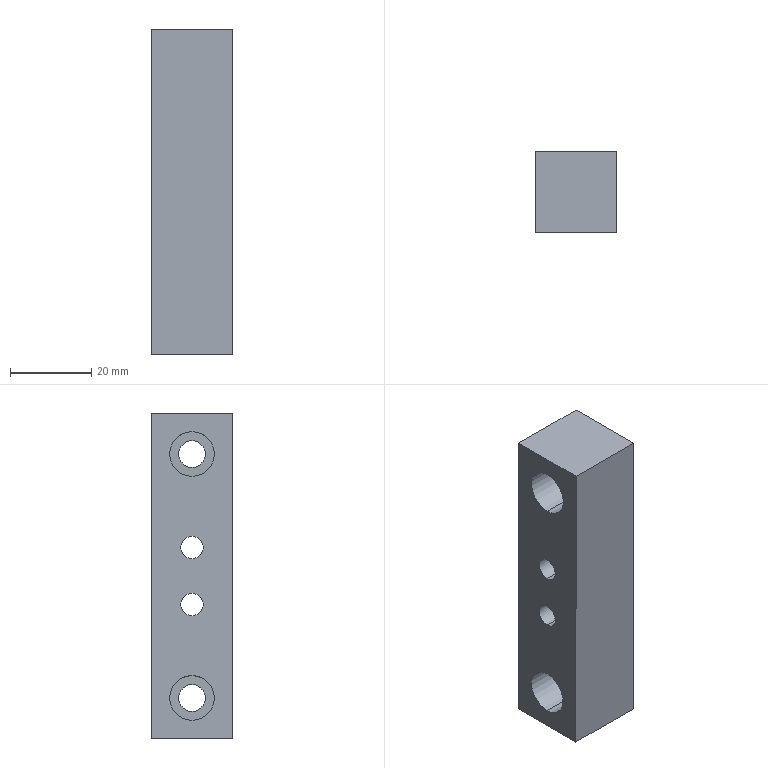Component | SolidWorks | ArmRotationCylinderConnectionBlock-1 | 1 solid | 26 faces | box 20.09 x 20 x 80.02 mm | volume 27354 mm3 | cylinder 16 | plane 10 | commonest cylinder face diameters 10 x4 5.5 x4 11 x4 6.6 x4
build123d program:
from build123d import *

# Parameters (mm, degrees)
SKETCH1_W                                       = 20
SKETCH1_H                                       = 80
BOSS_EXTRUDE1_DEPTH                             = 20
M6_HEX_SOCKET_HEAD_CAP_SCREW_CBORE1_D           = 6.6
M6_HEX_SOCKET_HEAD_CAP_SCREW_CBORE1_DEPTH       = 21
M6_HEX_SOCKET_HEAD_CAP_SCREW_CBORE1_CBORE_D     = 11
M6_HEX_SOCKET_HEAD_CAP_SCREW_CBORE1_CBORE_DEPTH = 14
M6_HEX_SOCKET_HEAD_CAP_SCREW_CBORE1_TIP         = 1.983
M5_HEX_SOCKET_HEAD_CAP_SCREW_CBORE1_D           = 5.5
M5_HEX_SOCKET_HEAD_CAP_SCREW_CBORE1_CBORE_D     = 10
M5_HEX_SOCKET_HEAD_CAP_SCREW_CBORE1_CBORE_DEPTH = 5.7


with BuildPart() as part:
    # Sketch1 → Boss-Extrude1 (new body)
    with BuildSketch(Plane(origin=(0, 0, 0), x_dir=(1, 0, 0), z_dir=(0, 1, 0))):
        Rectangle(SKETCH1_W, SKETCH1_H)
    extrude(amount=BOSS_EXTRUDE1_DEPTH)

    # M6 Hex Socket Head Cap Screw CBORE1
    with Locations(Plane.ZY.offset(10)):
        with Locations((-30, 10), (30, 10)):
            CounterBoreHole(M6_HEX_SOCKET_HEAD_CAP_SCREW_CBORE1_D / 2, M6_HEX_SOCKET_HEAD_CAP_SCREW_CBORE1_CBORE_D / 2, M6_HEX_SOCKET_HEAD_CAP_SCREW_CBORE1_CBORE_DEPTH, depth=M6_HEX_SOCKET_HEAD_CAP_SCREW_CBORE1_DEPTH)
            with Locations((0, 0, -(M6_HEX_SOCKET_HEAD_CAP_SCREW_CBORE1_DEPTH + M6_HEX_SOCKET_HEAD_CAP_SCREW_CBORE1_TIP / 2))):  # 118° drill point
                Cone(0, M6_HEX_SOCKET_HEAD_CAP_SCREW_CBORE1_D / 2, M6_HEX_SOCKET_HEAD_CAP_SCREW_CBORE1_TIP, mode=Mode.SUBTRACT)

    # M5 Hex Socket Head Cap Screw CBORE1 (through all)
    with Locations(Plane(origin=(10, 0, 0), x_dir=(0, 0, -1), z_dir=(1, 0, 0))):
        with Locations((-7, 10), (7, 10)):
            CounterBoreHole(M5_HEX_SOCKET_HEAD_CAP_SCREW_CBORE1_D / 2, M5_HEX_SOCKET_HEAD_CAP_SCREW_CBORE1_CBORE_D / 2, M5_HEX_SOCKET_HEAD_CAP_SCREW_CBORE1_CBORE_DEPTH)


solid = part.part

# Placed as in the assembly
solid = solid.moved(Location((-90.542, 904.54, 1109.715), (0, 0.0619, 0)))
STEP:
#1=COLOUR_RGB('',0.7922,0.8196,0.9333);
#2=FILL_AREA_STYLE_COLOUR('',#1);
#3=FILL_AREA_STYLE('',(#2));
#4=SURFACE_STYLE_FILL_AREA(#3);
#5=SURFACE_SIDE_STYLE('',(#4));
#6=SURFACE_STYLE_USAGE(.BOTH.,#5);
#7=PRESENTATION_STYLE_ASSIGNMENT((#6));
#8=CARTESIAN_POINT('',(-3.395,36.006,44.162));
#9=VERTEX_POINT('',#8);
#10=CARTESIAN_POINT('',(-3.395,36.006,43.768));
#11=VERTEX_POINT('',#10);
#12=CARTESIAN_POINT('',(-3.395,36.006,43.965));
#13=DIRECTION('',(1.,0.,-0.00108));
#14=DIRECTION('',(-0.00108,0.,-1.));
#15=AXIS2_PLACEMENT_3D('',#12,#13,#14);
#16=CIRCLE('',#15,0.1969);
#17=EDGE_CURVE('',#9,#11,#16,.T.);
#18=ORIENTED_EDGE('',*,*,#17,.F.);
#19=CARTESIAN_POINT('',(-3.17,36.006,44.162));
#20=VERTEX_POINT('',#19);
#21=CARTESIAN_POINT('',(-3.17,36.006,44.162));
#22=DIRECTION('',(1.,0.,-0.00108));
#23=VECTOR('',#22,39.37);
#24=LINE('',#21,#23);
#25=EDGE_CURVE('',#9,#20,#24,.T.);
#26=ORIENTED_EDGE('',*,*,#25,.T.);
#27=CARTESIAN_POINT('',(-3.171,36.006,43.768));
#28=VERTEX_POINT('',#27);
#29=CARTESIAN_POINT('',(-3.171,36.006,43.965));
#30=DIRECTION('',(1.,0.,-0.00108));
#31=DIRECTION('',(-0.00108,0.,-1.));
#32=AXIS2_PLACEMENT_3D('',#29,#30,#31);
#33=CIRCLE('',#32,0.1969);
#34=EDGE_CURVE('',#20,#28,#33,.T.);
#35=ORIENTED_EDGE('',*,*,#34,.T.);
#36=CARTESIAN_POINT('',(-3.171,36.006,43.768));
#37=DIRECTION('',(1.,0.,-0.00108));
#38=VECTOR('',#37,39.37);
#39=LINE('',#36,#38);
#40=EDGE_CURVE('',#11,#28,#39,.T.);
#41=ORIENTED_EDGE('',*,*,#40,.F.);
#42=EDGE_LOOP('',(#18,#26,#35,#41));
#43=FACE_OUTER_BOUND('',#42,.T.);
#44=CARTESIAN_POINT('',(-3.171,36.006,43.965));
#45=DIRECTION('',(1.,0.,-0.00108));
#46=DIRECTION('',(-0.00108,0.,-1.));
#47=AXIS2_PLACEMENT_3D('',#44,#45,#46);
#48=CYLINDRICAL_SURFACE('',#47,0.1969);
#49=ADVANCED_FACE('',(#43),#48,.F.);
#50=CARTESIAN_POINT('',(-3.958,36.006,44.074));
#51=VERTEX_POINT('',#50);
#52=CARTESIAN_POINT('',(-3.958,36.006,43.857));
#53=VERTEX_POINT('',#52);
#54=CARTESIAN_POINT('',(-3.958,36.006,43.966));
#55=DIRECTION('',(1.,0.,-0.00108));
#56=DIRECTION('',(-0.00108,0.,-1.));
#57=AXIS2_PLACEMENT_3D('',#54,#55,#56);
#58=CIRCLE('',#57,0.1083);
#59=EDGE_CURVE('',#51,#53,#58,.T.);
#60=ORIENTED_EDGE('',*,*,#59,.F.);
#61=CARTESIAN_POINT('',(-3.395,36.006,44.073));
#62=VERTEX_POINT('',#61);
#63=CARTESIAN_POINT('',(-3.171,36.006,44.073));
#64=DIRECTION('',(1.,0.,-0.00108));
#65=VECTOR('',#64,39.37);
#66=LINE('',#63,#65);
#67=EDGE_CURVE('',#51,#62,#66,.T.);
#68=ORIENTED_EDGE('',*,*,#67,.T.);
#69=CARTESIAN_POINT('',(-3.395,36.006,43.857));
#70=VERTEX_POINT('',#69);
#71=CARTESIAN_POINT('',(-3.395,36.006,43.965));
#72=DIRECTION('',(1.,0.,-0.00108));
#73=DIRECTION('',(-0.00108,0.,-1.));
#74=AXIS2_PLACEMENT_3D('',#71,#72,#73);
#75=CIRCLE('',#74,0.1083);
#76=EDGE_CURVE('',#62,#70,#75,.T.);
#77=ORIENTED_EDGE('',*,*,#76,.T.);
#78=CARTESIAN_POINT('',(-3.171,36.006,43.856));
#79=DIRECTION('',(1.,0.,-0.00108));
#80=VECTOR('',#79,39.37);
#81=LINE('',#78,#80);
#82=EDGE_CURVE('',#53,#70,#81,.T.);
#83=ORIENTED_EDGE('',*,*,#82,.F.);
#84=EDGE_LOOP('',(#60,#68,#77,#83));
#85=FACE_OUTER_BOUND('',#84,.T.);
#86=CARTESIAN_POINT('',(-3.171,36.006,43.965));
#87=DIRECTION('',(1.,0.,-0.00108));
#88=DIRECTION('',(-0.00108,0.,-1.));
#89=AXIS2_PLACEMENT_3D('',#86,#87,#88);
#90=CYLINDRICAL_SURFACE('',#89,0.1083);
#91=ADVANCED_FACE('',(#85),#90,.F.);
#92=CARTESIAN_POINT('',(-3.395,36.006,43.611));
#93=VERTEX_POINT('',#92);
#94=CARTESIAN_POINT('',(-3.396,36.006,43.217));
#95=VERTEX_POINT('',#94);
#96=CARTESIAN_POINT('',(-3.396,36.006,43.414));
#97=DIRECTION('',(1.,0.,-0.00108));
#98=DIRECTION('',(-0.00108,0.,-1.));
#99=AXIS2_PLACEMENT_3D('',#96,#97,#98);
#100=CIRCLE('',#99,0.1969);
#101=EDGE_CURVE('',#93,#95,#100,.T.);
#102=ORIENTED_EDGE('',*,*,#101,.F.);
#103=CARTESIAN_POINT('',(-3.171,36.006,43.61));
#104=VERTEX_POINT('',#103);
#105=CARTESIAN_POINT('',(-3.171,36.006,43.61));
#106=DIRECTION('',(1.,0.,-0.00108));
#107=VECTOR('',#106,39.37);
#108=LINE('',#105,#107);
#109=EDGE_CURVE('',#93,#104,#108,.T.);
#110=ORIENTED_EDGE('',*,*,#109,.T.);
#111=CARTESIAN_POINT('',(-3.171,36.006,43.217));
#112=VERTEX_POINT('',#111);
#113=CARTESIAN_POINT('',(-3.171,36.006,43.414));
#114=DIRECTION('',(1.,0.,-0.00108));
#115=DIRECTION('',(-0.00108,0.,-1.));
#116=AXIS2_PLACEMENT_3D('',#113,#114,#115);
#117=CIRCLE('',#116,0.1969);
#118=EDGE_CURVE('',#104,#112,#117,.T.);
#119=ORIENTED_EDGE('',*,*,#118,.T.);
#120=CARTESIAN_POINT('',(-3.171,36.006,43.217));
#121=DIRECTION('',(1.,0.,-0.00108));
#122=VECTOR('',#121,39.37);
#123=LINE('',#120,#122);
#124=EDGE_CURVE('',#95,#112,#123,.T.);
#125=ORIENTED_EDGE('',*,*,#124,.F.);
#126=EDGE_LOOP('',(#102,#110,#119,#125));
#127=FACE_OUTER_BOUND('',#126,.T.);
#128=CARTESIAN_POINT('',(-3.171,36.006,43.414));
#129=DIRECTION('',(1.,0.,-0.00108));
#130=DIRECTION('',(-0.00108,0.,-1.));
#131=AXIS2_PLACEMENT_3D('',#128,#129,#130);
#132=CYLINDRICAL_SURFACE('',#131,0.1969);
#133=ADVANCED_FACE('',(#127),#132,.F.);
#134=CARTESIAN_POINT('',(-3.959,36.006,43.523));
#135=VERTEX_POINT('',#134);
#136=CARTESIAN_POINT('',(-3.959,36.006,43.306));
#137=VERTEX_POINT('',#136);
#138=CARTESIAN_POINT('',(-3.959,36.006,43.414));
#139=DIRECTION('',(1.,0.,-0.00108));
#140=DIRECTION('',(-0.00108,0.,-1.));
#141=AXIS2_PLACEMENT_3D('',#138,#139,#140);
#142=CIRCLE('',#141,0.1083);
#143=EDGE_CURVE('',#135,#137,#142,.T.);
#144=ORIENTED_EDGE('',*,*,#143,.F.);
#145=CARTESIAN_POINT('',(-3.396,36.006,43.522));
#146=VERTEX_POINT('',#145);
#147=CARTESIAN_POINT('',(-3.171,36.006,43.522));
#148=DIRECTION('',(1.,0.,-0.00108));
#149=VECTOR('',#148,39.37);
#150=LINE('',#147,#149);
#151=EDGE_CURVE('',#135,#146,#150,.T.);
#152=ORIENTED_EDGE('',*,*,#151,.T.);
#153=CARTESIAN_POINT('',(-3.396,36.006,43.306));
#154=VERTEX_POINT('',#153);
#155=CARTESIAN_POINT('',(-3.396,36.006,43.414));
#156=DIRECTION('',(1.,0.,-0.00108));
#157=DIRECTION('',(-0.00108,0.,-1.));
#158=AXIS2_PLACEMENT_3D('',#155,#156,#157);
#159=CIRCLE('',#158,0.1083);
#160=EDGE_CURVE('',#146,#154,#159,.T.);
#161=ORIENTED_EDGE('',*,*,#160,.T.);
#162=CARTESIAN_POINT('',(-3.171,36.006,43.305));
#163=DIRECTION('',(1.,0.,-0.00108));
#164=VECTOR('',#163,39.37);
#165=LINE('',#162,#164);
#166=EDGE_CURVE('',#137,#154,#165,.T.);
#167=ORIENTED_EDGE('',*,*,#166,.F.);
#168=EDGE_LOOP('',(#144,#152,#161,#167));
#169=FACE_OUTER_BOUND('',#168,.T.);
#170=CARTESIAN_POINT('',(-3.171,36.006,43.414));
#171=DIRECTION('',(1.,0.,-0.00108));
#172=DIRECTION('',(-0.00108,0.,-1.));
#173=AXIS2_PLACEMENT_3D('',#170,#171,#172);
#174=CYLINDRICAL_SURFACE('',#173,0.1083);
#175=ADVANCED_FACE('',(#169),#174,.F.);
#176=CARTESIAN_POINT('',(-3.409,36.006,42.292));
#177=VERTEX_POINT('',#176);
#178=CARTESIAN_POINT('',(-3.408,36.006,42.725));
#179=VERTEX_POINT('',#178);
#180=CARTESIAN_POINT('',(-3.408,36.006,42.508));
#181=DIRECTION('',(-1.,-0.,0.00108));
#182=DIRECTION('',(0.00108,0.,1.));
#183=AXIS2_PLACEMENT_3D('',#180,#181,#182);
#184=CIRCLE('',#183,0.2165);
#185=EDGE_CURVE('',#177,#179,#184,.T.);
#186=ORIENTED_EDGE('',*,*,#185,.F.);
#187=CARTESIAN_POINT('',(-3.96,36.006,42.292));
#188=VERTEX_POINT('',#187);
#189=CARTESIAN_POINT('',(-3.96,36.006,42.292));
#190=DIRECTION('',(-1.,-0.,0.00108));
#191=VECTOR('',#190,39.37);
#192=LINE('',#189,#191);
#193=EDGE_CURVE('',#177,#188,#192,.T.);
#194=ORIENTED_EDGE('',*,*,#193,.T.);
#195=CARTESIAN_POINT('',(-3.959,36.006,42.725));
#196=VERTEX_POINT('',#195);
#197=CARTESIAN_POINT('',(-3.96,36.006,42.509));
#198=DIRECTION('',(-1.,-0.,0.00108));
#199=DIRECTION('',(0.00108,0.,1.));
#200=AXIS2_PLACEMENT_3D('',#197,#198,#199);
#201=CIRCLE('',#200,0.2165);
#202=EDGE_CURVE('',#188,#196,#201,.T.);
#203=ORIENTED_EDGE('',*,*,#202,.T.);
#204=CARTESIAN_POINT('',(-3.959,36.006,42.725));
#205=DIRECTION('',(-1.,-0.,0.00108));
#206=VECTOR('',#205,39.37);
#207=LINE('',#204,#206);
#208=EDGE_CURVE('',#179,#196,#207,.T.);
#209=ORIENTED_EDGE('',*,*,#208,.F.);
#210=EDGE_LOOP('',(#186,#194,#203,#209));
#211=FACE_OUTER_BOUND('',#210,.T.);
#212=CARTESIAN_POINT('',(-3.96,36.006,42.509));
#213=DIRECTION('',(-1.,-0.,0.00108));
#214=DIRECTION('',(0.00108,0.,1.));
#215=AXIS2_PLACEMENT_3D('',#212,#213,#214);
#216=CYLINDRICAL_SURFACE('',#215,0.2165);
#217=ADVANCED_FACE('',(#211),#216,.F.);
#218=CARTESIAN_POINT('',(-3.172,36.006,42.378));
#219=VERTEX_POINT('',#218);
#220=CARTESIAN_POINT('',(-3.172,36.006,42.638));
#221=VERTEX_POINT('',#220);
#222=CARTESIAN_POINT('',(-3.172,36.006,42.508));
#223=DIRECTION('',(-1.,-0.,0.00108));
#224=DIRECTION('',(0.00108,0.,1.));
#225=AXIS2_PLACEMENT_3D('',#222,#223,#224);
#226=CIRCLE('',#225,0.1299);
#227=EDGE_CURVE('',#219,#221,#226,.T.);
#228=ORIENTED_EDGE('',*,*,#227,.F.);
#229=CARTESIAN_POINT('',(-3.409,36.006,42.378));
#230=VERTEX_POINT('',#229);
#231=CARTESIAN_POINT('',(-3.96,36.006,42.379));
#232=DIRECTION('',(-1.,-0.,0.00108));
#233=VECTOR('',#232,39.37);
#234=LINE('',#231,#233);
#235=EDGE_CURVE('',#219,#230,#234,.T.);
#236=ORIENTED_EDGE('',*,*,#235,.T.);
#237=CARTESIAN_POINT('',(-3.408,36.006,42.638));
#238=VERTEX_POINT('',#237);
#239=CARTESIAN_POINT('',(-3.408,36.006,42.508));
#240=DIRECTION('',(-1.,-0.,0.00108));
#241=DIRECTION('',(0.00108,0.,1.));
#242=AXIS2_PLACEMENT_3D('',#239,#240,#241);
#243=CIRCLE('',#242,0.1299);
#244=EDGE_CURVE('',#230,#238,#243,.T.);
#245=ORIENTED_EDGE('',*,*,#244,.T.);
#246=CARTESIAN_POINT('',(-3.959,36.006,42.639));
#247=DIRECTION('',(-1.,-0.,0.00108));
#248=VECTOR('',#247,39.37);
#249=LINE('',#246,#248);
#250=EDGE_CURVE('',#221,#238,#249,.T.);
#251=ORIENTED_EDGE('',*,*,#250,.F.);
#252=EDGE_LOOP('',(#228,#236,#245,#251));
#253=FACE_OUTER_BOUND('',#252,.T.);
#254=CARTESIAN_POINT('',(-3.96,36.006,42.509));
#255=DIRECTION('',(-1.,-0.,0.00108));
#256=DIRECTION('',(0.00108,0.,1.));
#257=AXIS2_PLACEMENT_3D('',#254,#255,#256);
#258=CYLINDRICAL_SURFACE('',#257,0.1299);
#259=ADVANCED_FACE('',(#253),#258,.F.);
#260=CARTESIAN_POINT('',(-3.406,36.006,44.654));
#261=VERTEX_POINT('',#260);
#262=CARTESIAN_POINT('',(-3.406,36.006,45.087));
#263=VERTEX_POINT('',#262);
#264=CARTESIAN_POINT('',(-3.406,36.006,44.871));
#265=DIRECTION('',(-1.,-0.,0.00108));
#266=DIRECTION('',(0.00108,0.,1.));
#267=AXIS2_PLACEMENT_3D('',#264,#265,#266);
#268=CIRCLE('',#267,0.2165);
#269=EDGE_CURVE('',#261,#263,#268,.T.);
#270=ORIENTED_EDGE('',*,*,#269,.F.);
#271=CARTESIAN_POINT('',(-3.957,36.006,44.655));
#272=VERTEX_POINT('',#271);
#273=CARTESIAN_POINT('',(-3.957,36.006,44.655));
#274=DIRECTION('',(-1.,-0.,0.00108));
#275=VECTOR('',#274,39.37);
#276=LINE('',#273,#275);
#277=EDGE_CURVE('',#261,#272,#276,.T.);
#278=ORIENTED_EDGE('',*,*,#277,.T.);
#279=CARTESIAN_POINT('',(-3.957,36.006,45.088));
#280=VERTEX_POINT('',#279);
#281=CARTESIAN_POINT('',(-3.957,36.006,44.871));
#282=DIRECTION('',(-1.,-0.,0.00108));
#283=DIRECTION('',(0.00108,0.,1.));
#284=AXIS2_PLACEMENT_3D('',#281,#282,#283);
#285=CIRCLE('',#284,0.2165);
#286=EDGE_CURVE('',#272,#280,#285,.T.);
#287=ORIENTED_EDGE('',*,*,#286,.T.);
#288=CARTESIAN_POINT('',(-3.957,36.006,45.088));
#289=DIRECTION('',(-1.,-0.,0.00108));
#290=VECTOR('',#289,39.37);
#291=LINE('',#288,#290);
#292=EDGE_CURVE('',#263,#280,#291,.T.);
#293=ORIENTED_EDGE('',*,*,#292,.F.);
#294=EDGE_LOOP('',(#270,#278,#287,#293));
#295=FACE_OUTER_BOUND('',#294,.T.);
#296=CARTESIAN_POINT('',(-3.957,36.006,44.871));
#297=DIRECTION('',(-1.,-0.,0.00108));
#298=DIRECTION('',(0.00108,0.,1.));
#299=AXIS2_PLACEMENT_3D('',#296,#297,#298);
#300=CYLINDRICAL_SURFACE('',#299,0.2165);
#301=ADVANCED_FACE('',(#295),#300,.F.);
#302=CARTESIAN_POINT('',(-3.17,36.006,44.74));
#303=VERTEX_POINT('',#302);
#304=CARTESIAN_POINT('',(-3.17,36.006,45.));
#305=VERTEX_POINT('',#304);
#306=CARTESIAN_POINT('',(-3.17,36.006,44.87));
#307=DIRECTION('',(-1.,-0.,0.00108));
#308=DIRECTION('',(0.00108,0.,1.));
#309=AXIS2_PLACEMENT_3D('',#306,#307,#308);
#310=CIRCLE('',#309,0.1299);
#311=EDGE_CURVE('',#303,#305,#310,.T.);
#312=ORIENTED_EDGE('',*,*,#311,.F.);
#313=CARTESIAN_POINT('',(-3.406,36.006,44.741));
#314=VERTEX_POINT('',#313);
#315=CARTESIAN_POINT('',(-3.957,36.006,44.741));
#316=DIRECTION('',(-1.,-0.,0.00108));
#317=VECTOR('',#316,39.37);
#318=LINE('',#315,#317);
#319=EDGE_CURVE('',#303,#314,#318,.T.);
#320=ORIENTED_EDGE('',*,*,#319,.T.);
#321=CARTESIAN_POINT('',(-3.406,36.006,45.));
#322=VERTEX_POINT('',#321);
#323=CARTESIAN_POINT('',(-3.406,36.006,44.871));
#324=DIRECTION('',(-1.,-0.,0.00108));
#325=DIRECTION('',(0.00108,0.,1.));
#326=AXIS2_PLACEMENT_3D('',#323,#324,#325);
#327=CIRCLE('',#326,0.1299);
#328=EDGE_CURVE('',#314,#322,#327,.T.);
#329=ORIENTED_EDGE('',*,*,#328,.T.);
#330=CARTESIAN_POINT('',(-3.957,36.006,45.001));
#331=DIRECTION('',(-1.,-0.,0.00108));
#332=VECTOR('',#331,39.37);
#333=LINE('',#330,#332);
#334=EDGE_CURVE('',#305,#322,#333,.T.);
#335=ORIENTED_EDGE('',*,*,#334,.F.);
#336=EDGE_LOOP('',(#312,#320,#329,#335));
#337=FACE_OUTER_BOUND('',#336,.T.);
#338=CARTESIAN_POINT('',(-3.957,36.006,44.871));
#339=DIRECTION('',(-1.,-0.,0.00108));
#340=DIRECTION('',(0.00108,0.,1.));
#341=AXIS2_PLACEMENT_3D('',#338,#339,#340);
#342=CYLINDRICAL_SURFACE('',#341,0.1299);
#343=ADVANCED_FACE('',(#337),#342,.F.);
#344=CARTESIAN_POINT('',(-3.171,36.006,43.965));
#345=DIRECTION('',(1.,0.,-0.00108));
#346=DIRECTION('',(-0.00108,0.,-1.));
#347=AXIS2_PLACEMENT_3D('',#344,#345,#346);
#348=CIRCLE('',#347,0.1969);
#349=EDGE_CURVE('',#28,#20,#348,.T.);
#350=ORIENTED_EDGE('',*,*,#349,.F.);
#351=ORIENTED_EDGE('',*,*,#34,.F.);
#352=EDGE_LOOP('',(#350,#351));
#353=FACE_BOUND('',#352,.T.);
#354=CARTESIAN_POINT('',(-3.171,36.006,43.414));
#355=DIRECTION('',(1.,0.,-0.00108));
#356=DIRECTION('',(-0.00108,0.,-1.));
#357=AXIS2_PLACEMENT_3D('',#354,#355,#356);
#358=CIRCLE('',#357,0.1969);
#359=EDGE_CURVE('',#112,#104,#358,.T.);
#360=ORIENTED_EDGE('',*,*,#359,.F.);
#361=ORIENTED_EDGE('',*,*,#118,.F.);
#362=EDGE_LOOP('',(#360,#361));
#363=FACE_BOUND('',#362,.T.);
#364=CARTESIAN_POINT('',(-3.172,36.006,42.508));
#365=DIRECTION('',(-1.,-0.,0.00108));
#366=DIRECTION('',(0.00108,0.,1.));
#367=AXIS2_PLACEMENT_3D('',#364,#365,#366);
#368=CIRCLE('',#367,0.1299);
#369=EDGE_CURVE('',#221,#219,#368,.T.);
#370=ORIENTED_EDGE('',*,*,#369,.T.);
#371=ORIENTED_EDGE('',*,*,#227,.T.);
#372=EDGE_LOOP('',(#370,#371));
#373=FACE_BOUND('',#372,.T.);
#374=CARTESIAN_POINT('',(-3.17,36.006,44.87));
#375=DIRECTION('',(-1.,-0.,0.00108));
#376=DIRECTION('',(0.00108,0.,1.));
#377=AXIS2_PLACEMENT_3D('',#374,#375,#376);
#378=CIRCLE('',#377,0.1299);
#379=EDGE_CURVE('',#305,#303,#378,.T.);
#380=ORIENTED_EDGE('',*,*,#379,.T.);
#381=ORIENTED_EDGE('',*,*,#311,.T.);
#382=EDGE_LOOP('',(#380,#381));
#383=FACE_BOUND('',#382,.T.);
#384=CARTESIAN_POINT('',(-3.169,35.612,45.264));
#385=VERTEX_POINT('',#384);
#386=CARTESIAN_POINT('',(-3.173,35.612,42.114));
#387=VERTEX_POINT('',#386);
#388=CARTESIAN_POINT('',(-3.169,35.612,45.264));
#389=DIRECTION('',(-0.00108,-0.,-1.));
#390=VECTOR('',#389,39.37);
#391=LINE('',#388,#390);
#392=EDGE_CURVE('',#385,#387,#391,.T.);
#393=ORIENTED_EDGE('',*,*,#392,.T.);
#394=CARTESIAN_POINT('',(-3.173,36.399,42.114));
#395=VERTEX_POINT('',#394);
#396=CARTESIAN_POINT('',(-3.173,36.399,42.114));
#397=DIRECTION('',(0.,-1.,0.));
#398=VECTOR('',#397,39.37);
#399=LINE('',#396,#398);
#400=EDGE_CURVE('',#395,#387,#399,.T.);
#401=ORIENTED_EDGE('',*,*,#400,.F.);
#402=CARTESIAN_POINT('',(-3.169,36.399,45.264));
#403=VERTEX_POINT('',#402);
#404=CARTESIAN_POINT('',(-3.169,36.399,45.264));
#405=DIRECTION('',(-0.00108,-0.,-1.));
#406=VECTOR('',#405,39.37);
#407=LINE('',#404,#406);
#408=EDGE_CURVE('',#403,#395,#407,.T.);
#409=ORIENTED_EDGE('',*,*,#408,.F.);
#410=CARTESIAN_POINT('',(-3.169,36.399,45.264));
#411=DIRECTION('',(0.,-1.,0.));
#412=VECTOR('',#411,39.37);
#413=LINE('',#410,#412);
#414=EDGE_CURVE('',#403,#385,#413,.T.);
#415=ORIENTED_EDGE('',*,*,#414,.T.);
#416=EDGE_LOOP('',(#393,#401,#409,#415));
#417=FACE_OUTER_BOUND('',#416,.T.);
#418=CARTESIAN_POINT('',(-3.169,36.399,45.264));
#419=DIRECTION('',(-1.,-0.,0.00108));
#420=DIRECTION('',(0.00108,0.,1.));
#421=AXIS2_PLACEMENT_3D('',#418,#419,#420);
#422=PLANE('',#421);
#423=ADVANCED_FACE('',(#353,#363,#373,#383,#417),#422,.F.);
#424=CARTESIAN_POINT('',(-3.96,35.612,42.115));
#425=VERTEX_POINT('',#424);
#426=CARTESIAN_POINT('',(-3.96,35.612,42.115));
#427=DIRECTION('',(-1.,-0.,0.00108));
#428=VECTOR('',#427,39.37);
#429=LINE('',#426,#428);
#430=EDGE_CURVE('',#387,#425,#429,.T.);
#431=ORIENTED_EDGE('',*,*,#430,.T.);
#432=CARTESIAN_POINT('',(-3.96,36.399,42.115));
#433=VERTEX_POINT('',#432);
#434=CARTESIAN_POINT('',(-3.96,36.399,42.115));
#435=DIRECTION('',(0.,-1.,0.));
#436=VECTOR('',#435,39.37);
#437=LINE('',#434,#436);
#438=EDGE_CURVE('',#433,#425,#437,.T.);
#439=ORIENTED_EDGE('',*,*,#438,.F.);
#440=CARTESIAN_POINT('',(-3.96,36.399,42.115));
#441=DIRECTION('',(-1.,-0.,0.00108));
#442=VECTOR('',#441,39.37);
#443=LINE('',#440,#442);
#444=EDGE_CURVE('',#395,#433,#443,.T.);
#445=ORIENTED_EDGE('',*,*,#444,.F.);
#446=ORIENTED_EDGE('',*,*,#400,.T.);
#447=EDGE_LOOP('',(#431,#439,#445,#446));
#448=FACE_OUTER_BOUND('',#447,.T.);
#449=CARTESIAN_POINT('',(-3.96,36.399,42.115));
#450=DIRECTION('',(0.00108,0.,1.));
#451=DIRECTION('',(1.,0.,-0.00108));
#452=AXIS2_PLACEMENT_3D('',#449,#450,#451);
#453=PLANE('',#452);
#454=ADVANCED_FACE('',(#448),#453,.F.);
#455=CARTESIAN_POINT('',(-3.958,36.006,43.966));
#456=DIRECTION('',(1.,0.,-0.00108));
#457=DIRECTION('',(-0.00108,0.,-1.));
#458=AXIS2_PLACEMENT_3D('',#455,#456,#457);
#459=CIRCLE('',#458,0.1083);
#460=EDGE_CURVE('',#53,#51,#459,.T.);
#461=ORIENTED_EDGE('',*,*,#460,.T.);
#462=ORIENTED_EDGE('',*,*,#59,.T.);
#463=EDGE_LOOP('',(#461,#462));
#464=FACE_BOUND('',#463,.T.);
#465=CARTESIAN_POINT('',(-3.959,36.006,43.414));
#466=DIRECTION('',(1.,0.,-0.00108));
#467=DIRECTION('',(-0.00108,0.,-1.));
#468=AXIS2_PLACEMENT_3D('',#465,#466,#467);
#469=CIRCLE('',#468,0.1083);
#470=EDGE_CURVE('',#137,#135,#469,.T.);
#471=ORIENTED_EDGE('',*,*,#470,.T.);
#472=ORIENTED_EDGE('',*,*,#143,.T.);
#473=EDGE_LOOP('',(#471,#472));
#474=FACE_BOUND('',#473,.T.);
#475=CARTESIAN_POINT('',(-3.96,36.006,42.509));
#476=DIRECTION('',(-1.,-0.,0.00108));
#477=DIRECTION('',(0.00108,0.,1.));
#478=AXIS2_PLACEMENT_3D('',#475,#476,#477);
#479=CIRCLE('',#478,0.2165);
#480=EDGE_CURVE('',#196,#188,#479,.T.);
#481=ORIENTED_EDGE('',*,*,#480,.F.);
#482=ORIENTED_EDGE('',*,*,#202,.F.);
#483=EDGE_LOOP('',(#481,#482));
#484=FACE_BOUND('',#483,.T.);
#485=CARTESIAN_POINT('',(-3.957,36.006,44.871));
#486=DIRECTION('',(-1.,-0.,0.00108));
#487=DIRECTION('',(0.00108,0.,1.));
#488=AXIS2_PLACEMENT_3D('',#485,#486,#487);
#489=CIRCLE('',#488,0.2165);
#490=EDGE_CURVE('',#280,#272,#489,.T.);
#491=ORIENTED_EDGE('',*,*,#490,.F.);
#492=ORIENTED_EDGE('',*,*,#286,.F.);
#493=EDGE_LOOP('',(#491,#492));
#494=FACE_BOUND('',#493,.T.);
#495=CARTESIAN_POINT('',(-3.957,35.612,45.265));
#496=VERTEX_POINT('',#495);
#497=CARTESIAN_POINT('',(-3.957,35.612,45.265));
#498=DIRECTION('',(0.00108,0.,1.));
#499=VECTOR('',#498,39.37);
#500=LINE('',#497,#499);
#501=EDGE_CURVE('',#425,#496,#500,.T.);
#502=ORIENTED_EDGE('',*,*,#501,.T.);
#503=CARTESIAN_POINT('',(-3.957,36.399,45.265));
#504=VERTEX_POINT('',#503);
#505=CARTESIAN_POINT('',(-3.957,36.399,45.265));
#506=DIRECTION('',(0.,-1.,0.));
#507=VECTOR('',#506,39.37);
#508=LINE('',#505,#507);
#509=EDGE_CURVE('',#504,#496,#508,.T.);
#510=ORIENTED_EDGE('',*,*,#509,.F.);
#511=CARTESIAN_POINT('',(-3.957,36.399,45.265));
#512=DIRECTION('',(0.00108,0.,1.));
#513=VECTOR('',#512,39.37);
#514=LINE('',#511,#513);
#515=EDGE_CURVE('',#433,#504,#514,.T.);
#516=ORIENTED_EDGE('',*,*,#515,.F.);
#517=ORIENTED_EDGE('',*,*,#438,.T.);
#518=EDGE_LOOP('',(#502,#510,#516,#517));
#519=FACE_OUTER_BOUND('',#518,.T.);
#520=CARTESIAN_POINT('',(-3.957,36.399,45.265));
#521=DIRECTION('',(1.,0.,-0.00108));
#522=DIRECTION('',(-0.00108,-0.,-1.));
#523=AXIS2_PLACEMENT_3D('',#520,#521,#522);
#524=PLANE('',#523);
#525=ADVANCED_FACE('',(#464,#474,#484,#494,#519),#524,.F.);
#526=CARTESIAN_POINT('',(-3.957,35.612,45.265));
#527=DIRECTION('',(1.,0.,-0.00108));
#528=VECTOR('',#527,39.37);
#529=LINE('',#526,#528);
#530=EDGE_CURVE('',#496,#385,#529,.T.);
#531=ORIENTED_EDGE('',*,*,#530,.T.);
#532=ORIENTED_EDGE('',*,*,#414,.F.);
#533=CARTESIAN_POINT('',(-3.957,36.399,45.265));
#534=DIRECTION('',(1.,0.,-0.00108));
#535=VECTOR('',#534,39.37);
#536=LINE('',#533,#535);
#537=EDGE_CURVE('',#504,#403,#536,.T.);
#538=ORIENTED_EDGE('',*,*,#537,.F.);
#539=ORIENTED_EDGE('',*,*,#509,.T.);
#540=EDGE_LOOP('',(#531,#532,#538,#539));
#541=FACE_OUTER_BOUND('',#540,.T.);
#542=CARTESIAN_POINT('',(-3.957,36.399,45.265));
#543=DIRECTION('',(-0.00108,-0.,-1.));
#544=DIRECTION('',(-1.,-0.,0.00108));
#545=AXIS2_PLACEMENT_3D('',#542,#543,#544);
#546=PLANE('',#545);
#547=ADVANCED_FACE('',(#541),#546,.F.);
#548=ORIENTED_EDGE('',*,*,#408,.T.);
#549=ORIENTED_EDGE('',*,*,#444,.T.);
#550=ORIENTED_EDGE('',*,*,#515,.T.);
#551=ORIENTED_EDGE('',*,*,#537,.T.);
#552=EDGE_LOOP('',(#548,#549,#550,#551));
#553=FACE_OUTER_BOUND('',#552,.T.);
#554=CARTESIAN_POINT('',(-3.565,36.399,43.69));
#555=DIRECTION('',(0.,-1.,0.));
#556=DIRECTION('',(-0.00108,-0.,-1.));
#557=AXIS2_PLACEMENT_3D('',#554,#555,#556);
#558=PLANE('',#557);
#559=ADVANCED_FACE('',(#553),#558,.F.);
#560=ORIENTED_EDGE('',*,*,#392,.F.);
#561=ORIENTED_EDGE('',*,*,#530,.F.);
#562=ORIENTED_EDGE('',*,*,#501,.F.);
#563=ORIENTED_EDGE('',*,*,#430,.F.);
#564=EDGE_LOOP('',(#560,#561,#562,#563));
#565=FACE_OUTER_BOUND('',#564,.T.);
#566=CARTESIAN_POINT('',(-3.565,35.612,43.69));
#567=DIRECTION('',(0.,-1.,0.));
#568=DIRECTION('',(-0.00108,-0.,-1.));
#569=AXIS2_PLACEMENT_3D('',#566,#567,#568);
#570=PLANE('',#569);
#571=ADVANCED_FACE('',(#565),#570,.T.);
#572=ORIENTED_EDGE('',*,*,#319,.F.);
#573=ORIENTED_EDGE('',*,*,#379,.F.);
#574=ORIENTED_EDGE('',*,*,#334,.T.);
#575=CARTESIAN_POINT('',(-3.406,36.006,44.871));
#576=DIRECTION('',(-1.,-0.,0.00108));
#577=DIRECTION('',(0.00108,0.,1.));
#578=AXIS2_PLACEMENT_3D('',#575,#576,#577);
#579=CIRCLE('',#578,0.1299);
#580=EDGE_CURVE('',#322,#314,#579,.T.);
#581=ORIENTED_EDGE('',*,*,#580,.T.);
#582=EDGE_LOOP('',(#572,#573,#574,#581));
#583=FACE_OUTER_BOUND('',#582,.T.);
#584=CARTESIAN_POINT('',(-3.957,36.006,44.871));
#585=DIRECTION('',(-1.,-0.,0.00108));
#586=DIRECTION('',(0.00108,0.,1.));
#587=AXIS2_PLACEMENT_3D('',#584,#585,#586);
#588=CYLINDRICAL_SURFACE('',#587,0.1299);
#589=ADVANCED_FACE('',(#583),#588,.F.);
#590=ORIENTED_EDGE('',*,*,#580,.F.);
#591=ORIENTED_EDGE('',*,*,#328,.F.);
#592=EDGE_LOOP('',(#590,#591));
#593=FACE_BOUND('',#592,.T.);
#594=CARTESIAN_POINT('',(-3.406,36.006,44.871));
#595=DIRECTION('',(-1.,-0.,0.00108));
#596=DIRECTION('',(0.00108,0.,1.));
#597=AXIS2_PLACEMENT_3D('',#594,#595,#596);
#598=CIRCLE('',#597,0.2165);
#599=EDGE_CURVE('',#263,#261,#598,.T.);
#600=ORIENTED_EDGE('',*,*,#599,.T.);
#601=ORIENTED_EDGE('',*,*,#269,.T.);
#602=EDGE_LOOP('',(#600,#601));
#603=FACE_OUTER_BOUND('',#602,.T.);
#604=CARTESIAN_POINT('',(-3.406,36.135,44.871));
#605=DIRECTION('',(1.,0.,-0.00108));
#606=DIRECTION('',(-0.00108,-0.,-1.));
#607=AXIS2_PLACEMENT_3D('',#604,#605,#606);
#608=PLANE('',#607);
#609=ADVANCED_FACE('',(#593,#603),#608,.F.);
#610=ORIENTED_EDGE('',*,*,#277,.F.);
#611=ORIENTED_EDGE('',*,*,#599,.F.);
#612=ORIENTED_EDGE('',*,*,#292,.T.);
#613=ORIENTED_EDGE('',*,*,#490,.T.);
#614=EDGE_LOOP('',(#610,#611,#612,#613));
#615=FACE_OUTER_BOUND('',#614,.T.);
#616=CARTESIAN_POINT('',(-3.957,36.006,44.871));
#617=DIRECTION('',(-1.,-0.,0.00108));
#618=DIRECTION('',(0.00108,0.,1.));
#619=AXIS2_PLACEMENT_3D('',#616,#617,#618);
#620=CYLINDRICAL_SURFACE('',#619,0.2165);
#621=ADVANCED_FACE('',(#615),#620,.F.);
#622=ORIENTED_EDGE('',*,*,#235,.F.);
#623=ORIENTED_EDGE('',*,*,#369,.F.);
#624=ORIENTED_EDGE('',*,*,#250,.T.);
#625=CARTESIAN_POINT('',(-3.408,36.006,42.508));
#626=DIRECTION('',(-1.,-0.,0.00108));
#627=DIRECTION('',(0.00108,0.,1.));
#628=AXIS2_PLACEMENT_3D('',#625,#626,#627);
#629=CIRCLE('',#628,0.1299);
#630=EDGE_CURVE('',#238,#230,#629,.T.);
#631=ORIENTED_EDGE('',*,*,#630,.T.);
#632=EDGE_LOOP('',(#622,#623,#624,#631));
#633=FACE_OUTER_BOUND('',#632,.T.);
#634=CARTESIAN_POINT('',(-3.96,36.006,42.509));
#635=DIRECTION('',(-1.,-0.,0.00108));
#636=DIRECTION('',(0.00108,0.,1.));
#637=AXIS2_PLACEMENT_3D('',#634,#635,#636);
#638=CYLINDRICAL_SURFACE('',#637,0.1299);
#639=ADVANCED_FACE('',(#633),#638,.F.);
#640=ORIENTED_EDGE('',*,*,#630,.F.);
#641=ORIENTED_EDGE('',*,*,#244,.F.);
#642=EDGE_LOOP('',(#640,#641));
#643=FACE_BOUND('',#642,.T.);
#644=CARTESIAN_POINT('',(-3.408,36.006,42.508));
#645=DIRECTION('',(-1.,-0.,0.00108));
#646=DIRECTION('',(0.00108,0.,1.));
#647=AXIS2_PLACEMENT_3D('',#644,#645,#646);
#648=CIRCLE('',#647,0.2165);
#649=EDGE_CURVE('',#179,#177,#648,.T.);
#650=ORIENTED_EDGE('',*,*,#649,.T.);
#651=ORIENTED_EDGE('',*,*,#185,.T.);
#652=EDGE_LOOP('',(#650,#651));
#653=FACE_OUTER_BOUND('',#652,.T.);
#654=CARTESIAN_POINT('',(-3.408,36.135,42.508));
#655=DIRECTION('',(1.,0.,-0.00108));
#656=DIRECTION('',(-0.00108,-0.,-1.));
#657=AXIS2_PLACEMENT_3D('',#654,#655,#656);
#658=PLANE('',#657);
#659=ADVANCED_FACE('',(#643,#653),#658,.F.);
#660=ORIENTED_EDGE('',*,*,#193,.F.);
#661=ORIENTED_EDGE('',*,*,#649,.F.);
#662=ORIENTED_EDGE('',*,*,#208,.T.);
#663=ORIENTED_EDGE('',*,*,#480,.T.);
#664=EDGE_LOOP('',(#660,#661,#662,#663));
#665=FACE_OUTER_BOUND('',#664,.T.);
#666=CARTESIAN_POINT('',(-3.96,36.006,42.509));
#667=DIRECTION('',(-1.,-0.,0.00108));
#668=DIRECTION('',(0.00108,0.,1.));
#669=AXIS2_PLACEMENT_3D('',#666,#667,#668);
#670=CYLINDRICAL_SURFACE('',#669,0.2165);
#671=ADVANCED_FACE('',(#665),#670,.F.);
#672=ORIENTED_EDGE('',*,*,#151,.F.);
#673=ORIENTED_EDGE('',*,*,#470,.F.);
#674=ORIENTED_EDGE('',*,*,#166,.T.);
#675=CARTESIAN_POINT('',(-3.396,36.006,43.414));
#676=DIRECTION('',(1.,0.,-0.00108));
#677=DIRECTION('',(-0.00108,0.,-1.));
#678=AXIS2_PLACEMENT_3D('',#675,#676,#677);
#679=CIRCLE('',#678,0.1083);
#680=EDGE_CURVE('',#154,#146,#679,.T.);
#681=ORIENTED_EDGE('',*,*,#680,.T.);
#682=EDGE_LOOP('',(#672,#673,#674,#681));
#683=FACE_OUTER_BOUND('',#682,.T.);
#684=CARTESIAN_POINT('',(-3.171,36.006,43.414));
#685=DIRECTION('',(1.,0.,-0.00108));
#686=DIRECTION('',(-0.00108,0.,-1.));
#687=AXIS2_PLACEMENT_3D('',#684,#685,#686);
#688=CYLINDRICAL_SURFACE('',#687,0.1083);
#689=ADVANCED_FACE('',(#683),#688,.F.);
#690=ORIENTED_EDGE('',*,*,#680,.F.);
#691=ORIENTED_EDGE('',*,*,#160,.F.);
#692=EDGE_LOOP('',(#690,#691));
#693=FACE_BOUND('',#692,.T.);
#694=CARTESIAN_POINT('',(-3.396,36.006,43.414));
#695=DIRECTION('',(1.,0.,-0.00108));
#696=DIRECTION('',(-0.00108,0.,-1.));
#697=AXIS2_PLACEMENT_3D('',#694,#695,#696);
#698=CIRCLE('',#697,0.1969);
#699=EDGE_CURVE('',#95,#93,#698,.T.);
#700=ORIENTED_EDGE('',*,*,#699,.T.);
#701=ORIENTED_EDGE('',*,*,#101,.T.);
#702=EDGE_LOOP('',(#700,#701));
#703=FACE_OUTER_BOUND('',#702,.T.);
#704=CARTESIAN_POINT('',(-3.396,36.114,43.414));
#705=DIRECTION('',(-1.,-0.,0.00108));
#706=DIRECTION('',(0.00108,0.,1.));
#707=AXIS2_PLACEMENT_3D('',#704,#705,#706);
#708=PLANE('',#707);
#709=ADVANCED_FACE('',(#693,#703),#708,.F.);
#710=ORIENTED_EDGE('',*,*,#109,.F.);
#711=ORIENTED_EDGE('',*,*,#699,.F.);
#712=ORIENTED_EDGE('',*,*,#124,.T.);
#713=ORIENTED_EDGE('',*,*,#359,.T.);
#714=EDGE_LOOP('',(#710,#711,#712,#713));
#715=FACE_OUTER_BOUND('',#714,.T.);
#716=CARTESIAN_POINT('',(-3.171,36.006,43.414));
#717=DIRECTION('',(1.,0.,-0.00108));
#718=DIRECTION('',(-0.00108,0.,-1.));
#719=AXIS2_PLACEMENT_3D('',#716,#717,#718);
#720=CYLINDRICAL_SURFACE('',#719,0.1969);
#721=ADVANCED_FACE('',(#715),#720,.F.);
#722=ORIENTED_EDGE('',*,*,#67,.F.);
#723=ORIENTED_EDGE('',*,*,#460,.F.);
#724=ORIENTED_EDGE('',*,*,#82,.T.);
#725=CARTESIAN_POINT('',(-3.395,36.006,43.965));
#726=DIRECTION('',(1.,0.,-0.00108));
#727=DIRECTION('',(-0.00108,0.,-1.));
#728=AXIS2_PLACEMENT_3D('',#725,#726,#727);
#729=CIRCLE('',#728,0.1083);
#730=EDGE_CURVE('',#70,#62,#729,.T.);
#731=ORIENTED_EDGE('',*,*,#730,.T.);
#732=EDGE_LOOP('',(#722,#723,#724,#731));
#733=FACE_OUTER_BOUND('',#732,.T.);
#734=CARTESIAN_POINT('',(-3.171,36.006,43.965));
#735=DIRECTION('',(1.,0.,-0.00108));
#736=DIRECTION('',(-0.00108,0.,-1.));
#737=AXIS2_PLACEMENT_3D('',#734,#735,#736);
#738=CYLINDRICAL_SURFACE('',#737,0.1083);
#739=ADVANCED_FACE('',(#733),#738,.F.);
#740=ORIENTED_EDGE('',*,*,#730,.F.);
#741=ORIENTED_EDGE('',*,*,#76,.F.);
#742=EDGE_LOOP('',(#740,#741));
#743=FACE_BOUND('',#742,.T.);
#744=CARTESIAN_POINT('',(-3.395,36.006,43.965));
#745=DIRECTION('',(1.,0.,-0.00108));
#746=DIRECTION('',(-0.00108,0.,-1.));
#747=AXIS2_PLACEMENT_3D('',#744,#745,#746);
#748=CIRCLE('',#747,0.1969);
#749=EDGE_CURVE('',#11,#9,#748,.T.);
#750=ORIENTED_EDGE('',*,*,#749,.T.);
#751=ORIENTED_EDGE('',*,*,#17,.T.);
#752=EDGE_LOOP('',(#750,#751));
#753=FACE_OUTER_BOUND('',#752,.T.);
#754=CARTESIAN_POINT('',(-3.395,36.114,43.965));
#755=DIRECTION('',(-1.,-0.,0.00108));
#756=DIRECTION('',(0.00108,0.,1.));
#757=AXIS2_PLACEMENT_3D('',#754,#755,#756);
#758=PLANE('',#757);
#759=ADVANCED_FACE('',(#743,#753),#758,.F.);
#760=ORIENTED_EDGE('',*,*,#25,.F.);
#761=ORIENTED_EDGE('',*,*,#749,.F.);
#762=ORIENTED_EDGE('',*,*,#40,.T.);
#763=ORIENTED_EDGE('',*,*,#349,.T.);
#764=EDGE_LOOP('',(#760,#761,#762,#763));
#765=FACE_OUTER_BOUND('',#764,.T.);
#766=CARTESIAN_POINT('',(-3.171,36.006,43.965));
#767=DIRECTION('',(1.,0.,-0.00108));
#768=DIRECTION('',(-0.00108,0.,-1.));
#769=AXIS2_PLACEMENT_3D('',#766,#767,#768);
#770=CYLINDRICAL_SURFACE('',#769,0.1969);
#771=ADVANCED_FACE('',(#765),#770,.F.);
#772=CLOSED_SHELL('',(#49,#91,#133,#175,#217,#259,#301,#343,#423,#454,#525,#547,#559,#571,#589,#609,#621,#639,#659,#671,#689,#709,#721,#739,#759,#771));
#773=MANIFOLD_SOLID_BREP('',#772);
#774=STYLED_ITEM('',(#7),#773);
#775=(LENGTH_UNIT()NAMED_UNIT(*)SI_UNIT($,.METRE.));
#776=LENGTH_MEASURE_WITH_UNIT(LENGTH_MEASURE(0.0254),#775);
#777=DIMENSIONAL_EXPONENTS(1.,0.,0.,0.,0.,0.,0.);
#778=(CONVERSION_BASED_UNIT('',#776)LENGTH_UNIT()NAMED_UNIT(#777));
#779=UNCERTAINTY_MEASURE_WITH_UNIT(LENGTH_MEASURE(0.00001),#778,'','');
#780=(NAMED_UNIT(*)PLANE_ANGLE_UNIT()SI_UNIT($,.RADIAN.));
#781=(NAMED_UNIT(*)SI_UNIT($,.STERADIAN.)SOLID_ANGLE_UNIT());
#782=(GEOMETRIC_REPRESENTATION_CONTEXT(3)GLOBAL_UNCERTAINTY_ASSIGNED_CONTEXT((#779))GLOBAL_UNIT_ASSIGNED_CONTEXT((#778,#780,#781))REPRESENTATION_CONTEXT('',''));
#783=MECHANICAL_DESIGN_GEOMETRIC_PRESENTATION_REPRESENTATION('',(#774),#782);
#784=PRESENTATION_LAYER_ASSIGNMENT('','',(#774));
#785=CARTESIAN_POINT('',(0.,0.,0.));
#786=DIRECTION('',(0.,0.,1.));
#787=DIRECTION('',(1.,0.,0.));
#788=AXIS2_PLACEMENT_3D('',#785,#786,#787);
#789=(LENGTH_UNIT()NAMED_UNIT(*)SI_UNIT($,.METRE.));
#790=LENGTH_MEASURE_WITH_UNIT(LENGTH_MEASURE(0.0254),#789);
#791=DIMENSIONAL_EXPONENTS(1.,0.,0.,0.,0.,0.,0.);
#792=(CONVERSION_BASED_UNIT('',#790)LENGTH_UNIT()NAMED_UNIT(#791));
#793=UNCERTAINTY_MEASURE_WITH_UNIT(LENGTH_MEASURE(0.00001),#792,'','');
#794=(NAMED_UNIT(*)PLANE_ANGLE_UNIT()SI_UNIT($,.RADIAN.));
#795=(NAMED_UNIT(*)SI_UNIT($,.STERADIAN.)SOLID_ANGLE_UNIT());
#796=(GEOMETRIC_REPRESENTATION_CONTEXT(3)GLOBAL_UNCERTAINTY_ASSIGNED_CONTEXT((#793))GLOBAL_UNIT_ASSIGNED_CONTEXT((#792,#794,#795))REPRESENTATION_CONTEXT('',''));
#797=ADVANCED_BREP_SHAPE_REPRESENTATION('',(#773,#788),#796);